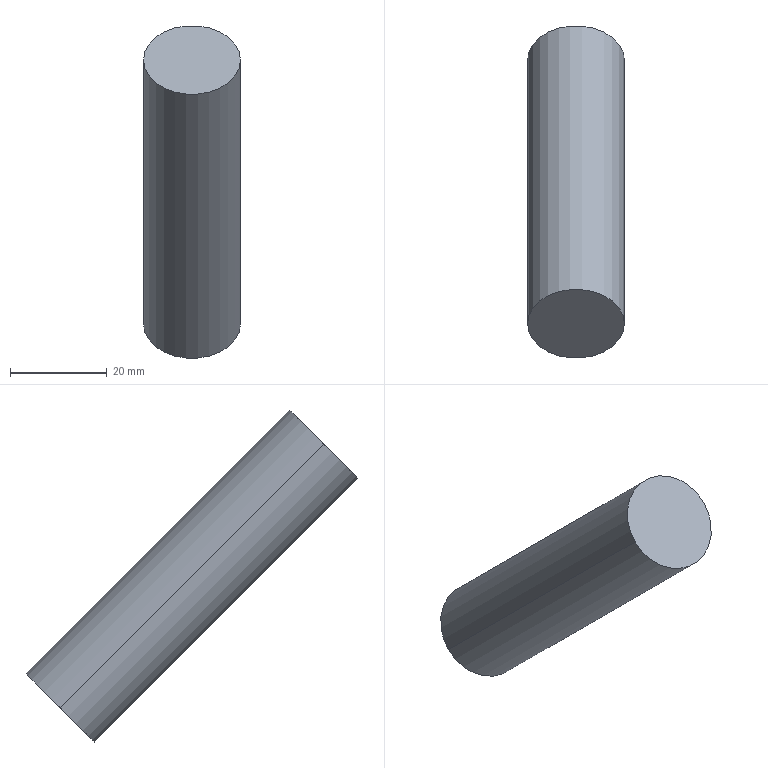Component | SolidWorks | Cylinder16X30-1 | 1 solid | 4 faces | box 20 x 68.59 x 68.59 mm | volume 24190 mm3 | cylinder 2 | plane 2 | commonest cylinder face diameters 20 x2
build123d program:
from build123d import *

# Parameters (mm, degrees)
SKETCH1_R      = 10
EXTRUDE1_DEPTH = 77


with BuildPart() as part:
    # Sketch1 → Extrude1 (new body)
    with BuildSketch(Plane(origin=(0, 0, 0), x_dir=(0, 0, -1), z_dir=(1, 0, 0))):
        Circle(SKETCH1_R)
    extrude(amount=EXTRUDE1_DEPTH)


solid = part.part

# Placed as in the assembly
solid = solid.moved(Location((44.323, 16.651, 28.684), (-45, 57.53, -90)))